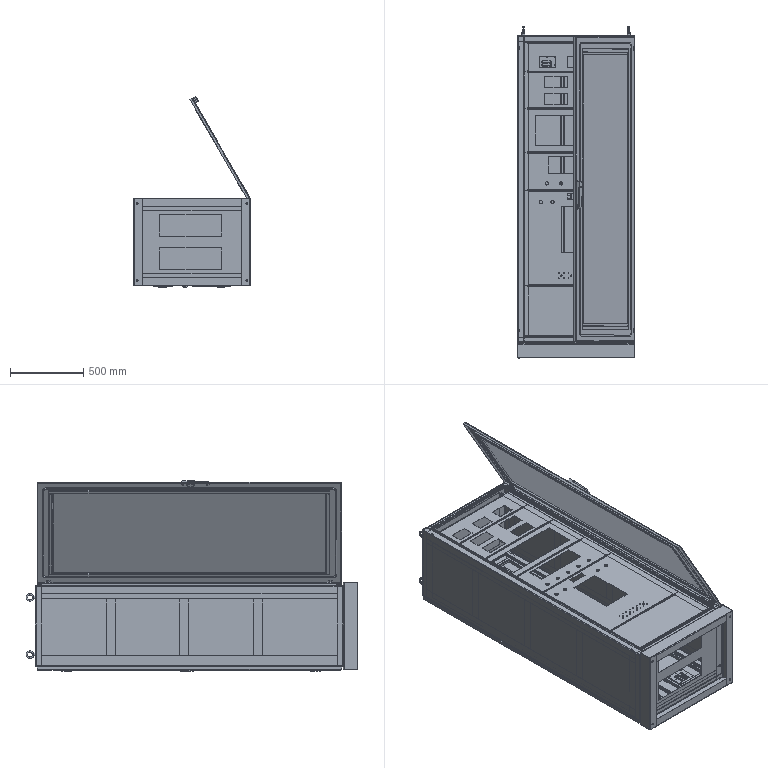Assembly | SolidWorks | mm | 69 component files | 69 solids | 2318 faces | box 801.74 x 2268 x 1304.71 mm | volume 31385291 mm3 | plane 1327 | cylinder 748 | torus 97 | sphere 64 | spline 46 | cone 36 | commonest cylinder face diameters 5 x100 7 x99 11 x91 4.5 x88 12.5 x48 3.2 x48 10 x48 2 x36
Bill of materials:
BaseFront-Rear | 2 |  | Long, thin-walled U-shaped channel with rounded inside bends. The base web runs past the ends of the two side walls at both ends.
BaseLeft-Right | 2 |  | Tall, thin-walled U or C channel with rounded bend corners. One side flange has two small round holes, one near each end.
Box | 2 | Plain Carbon Steel | Long, thin sheet panel with a C-shaped profile. A flat web has short flanges along both long edges, and each flange ends in a small hooked return lip.
CL201-M6-1 | 6 |  | Solid hinge-like block. An L-shaped body has two cylindrical knuckles with a shared pin bore at the two ends of one edge, a recessed gap between the knuckles, and a base leaf with two countersunk through holes and a chamfered edge.
CL201-M6-2 | 6 |  | Flat rectangular leaf plate with two round through holes. One edge thickens into a rounded knuckle lobe with a pin bore, as in a hinge leaf.
DoorLeftAndRightReinforcementBar | 6 | Malleable Cast Iron | Very long, slender, thin-walled channel. The end profile is a U shape with rounded bends and splayed straight legs.
DoorUpperAndLowerReinforcementBar | 2 | Malleable Cast Iron | Long, slender bar or channel. One end is rounded and the other end has a notched, C-like open profile. A recess or groove runs along its length.
FrontDoor | 1 | Malleable Cast Iron | Thin, flat rectangular frame plate with a large central rectangular cutout with small corner radii. A small rectangular slot and tiny holes sit near one long edge, and tiny holes are visible near the outer corners.
Glass | 1 | Plexiglas (TM) GS Acrylic Cast Sheet | Thin, plain, flat rectangular plate with no visible holes or cutouts.
MS829 | 1 | Cast Alloy Steel | Compact solid body with a stepped rectangular base. On one face is an elongated, tapered, raised paddle with a rounded end. On the opposite side is a protruding block with a cylindrical boss or pin. It looks like a lever or handle.
RubberPad | 1 | Silicone Rubber | Closed rectangular loop with rounded corners and a slender, thin cross-section, like a narrow rim or seal-shaped frame.
RearDoor1 | 1 | Malleable Cast Iron | Long, flat, thin rectangular sheet panel with shallow turned edges. One long edge has a small hooked return lip. Near each end is a small grid of perforation holes.
RearDoorUpperAndLowerReinforcementBar | 6 | Malleable Cast Iron | Long straight channel of uniform cross-section with an inverted-U profile (flat top, two parallel side legs, rounded outer corners), open along the bottom.
Vent | 4 | AISI 304 | Flat square plate with four parallel elongated louver-style formed openings in the middle and eight small round through-holes around the edge (corners and edge midpoints).
LiftingRingM12 | 4 |  | Ring-shaped eye with a round cross-section, joined to a cylindrical collar, with a smaller-diameter straight cylindrical shank coming out of the collar along the ring's radius.
LowerBaffle | 1 |  | Flat rectangular panel with two large rectangular cutouts stacked one above the other, four small holes near the side edges, and long formed flanges with short return lips along the top and bottom edges.
Panel1 | 1 | Malleable Cast Iron | Thin rectangular cover plate with three equal rectangular cutouts in a row, short downturned flanges along the two long edges, and small notches at the ends of the flanges.
Panel2 | 1 | Plain Carbon Steel | Thin rectangular cover plate with four rectangular cutouts in a 2x2 grid, short downturned flanges along the two long edges, and small notches where the flanges end.
Panel3 | 1 | Malleable Cast Iron | Thin rectangular frame-like plate with one large rectangular cutout in the middle, short downturned flanges along the two long edges, and notches where the flanges end.
Panel4 | 1 | Malleable Cast Iron | Thin rectangular cover plate with one rectangular cutout offset toward one long edge, a row of five equal round holes along the other long edge, and short downturned flanges along both long edges.
Panel5 | 1 | Malleable Cast Iron | Large thin rectangular plate with a tall rectangular cutout in the middle, a small rectangular slot above it, four round holes in a row near one edge, a pattern of small holes near the opposite edge, and very shallow downturned flanges along two edges.
Panel6 | 1 | Malleable Cast Iron | Plain thin rectangular plate with no openings, with short downturned flanges along the two long edges and notches where the flanges end.
PanelMountingBracket | 4 | Malleable Cast Iron | Long slender strip with an L-shaped (angle) cross-section, with a rounded inside bend between a wider leg and a narrower leg.
Lock818 | 1 |  | Small elongated part on a thin rectangular base plate. A raised block with rounded corners at one end slopes down to a long lower bar. A cylindrical post at the other end holds up a thin flat arm that runs back over the bar, parallel to it and spaced above it. A rounded protrusion sits on the underside.
RearDoor | 1 | Malleable Cast Iron | Long, narrow, thin rectangular plate or shallow tray with short edge returns along the perimeter, a rectangular slot near the middle of one long edge, and small groups of holes near each end.
SideBottomPlate | 2 | Plain Carbon Steel | Plain thin flat rectangular plate with no visible holes, cutouts or bends.
SideBottomPlateBracket | 6 | Malleable Cast Iron | Plain elongated flat rectangular strip or panel with no visible holes, cutouts or bends.
StiffenerPlate | 2 |  | Rectangular frame with a large central rectangular opening, narrow side bands each with two small round holes, and shallow return edges around the outer perimeter.
UpperBaffle | 1 |  | Flat rectangular panel with four small round corner holes. Top and bottom edges are formed into offset flanges with small lips, giving a C-like profile with hooked ends.
Mates:
1. coincident | StiffenerPlate-1 face at (-481.059, -83.54, -4140.526) dir (-1, 0, 0) | Box-1 face at (-481.059, 1976.46, -160.526) dir (1, 0, 0)
2. parallel | StiffenerPlate-1 face at (-4461.059, -83.54, 385.474) dir (0, 0, 1) | Box-1 face at (-433.059, 1976.46, -162.526) dir (0, 0, -1)
3. coincident | StiffenerPlate-1 face at (4294.941, -83.54, -160.526) dir (0, 0, -1) | Box-1 face at (-433.059, 1976.46, -160.526) dir (0, 0, 1)
4. coincident | StiffenerPlate-1 face at (214.919, -123.54, -84.019) dir (0, -1, 0) | Box-1 face at (-483.059, -123.54, -157.026) dir (0, -1, 0)
5. coincident | StiffenerPlate-1 face at (314.941, -83.54, 4365.474) dir (1, 0, 0) | Box-2 face at (314.941, -123.54, -160.526) dir (-1, 0, 0)
6. coincident | Box-1 face at (-433.059, 1976.46, -162.526) dir (0, 0, -1) | Box-2 face at (266.941, -123.54, -162.526) dir (0, 0, -1)
7. coincident | StiffenerPlate-1 face at (214.919, -123.54, -84.019) dir (0, -1, 0) | Box-2 face at (268.941, -123.54, -166.026) dir (0, -1, 0)
8. coincident | Box-1 face at (-481.059, 1976.46, -160.526) dir (1, 0, 0) | StiffenerPlate-2 face at (-481.059, 1936.46, 4365.474) dir (-1, 0, 0)
9. coincident | Box-2 face at (316.941, 1976.46, -157.026) dir (0, 1, 0) | StiffenerPlate-2 face at (214.919, 1976.46, 308.967) dir (0, 1, 0)
10. coincident | Box-2 face at (314.941, -123.54, 385.474) dir (0, 0, -1) | StiffenerPlate-2 face at (4294.941, 1936.46, 385.474) dir (0, 0, 1)
11. coincident | Box-1 face at (-481.059, 1976.46, 387.474) dir (0, 0, 1) | UpperBaffle-1 face at (316.941, 1930.46, 387.474) dir (0, 0, 1)
12. coincident | Box-1 face at (-483.059, 1976.46, -160.526) dir (-1, 0, 0) | UpperBaffle-1 face at (-483.059, 1972.96, -160.526) dir (-1, 0, 0)
13. coincident | Box-1 face at (-477.559, 1976.46, -162.526) dir (0, 1, 0) | UpperBaffle-1 face at (316.941, 1976.46, 387.474) dir (0, -1, 0)
14. concentric | UpperBaffle-1 face at (276.941, 1928.459, -82.526) dir (0, 1, 0) r 6.25 | LiftingRingM12-2 face at (276.941, 1953.46, -82.526) dir (0, 1, 0) r 6
15. coincident | UpperBaffle-1 face at (316.941, 1978.46, 387.474) dir (0, 1, 0) | LiftingRingM12-2 face at (276.941, 1978.46, -82.526) dir (0, -1, 0)
16. concentric | UpperBaffle-1 face at (276.941, 1928.459, 307.474) dir (0, 1, 0) r 6.25 | LiftingRingM12-1 face at (276.941, 1953.46, 307.474) dir (0, 1, 0) r 6
17. coincident | UpperBaffle-1 face at (316.941, 1978.46, 387.474) dir (0, 1, 0) | LiftingRingM12-1 face at (276.941, 1978.46, 307.474) dir (0, -1, 0)
18. concentric | UpperBaffle-1 face at (-443.059, 1928.459, 307.474) dir (0, 1, 0) r 6.25 | LiftingRingM12-4 face at (-443.059, 1953.46, 307.474) dir (0, 1, 0) r 6
19. coincident | UpperBaffle-1 face at (316.941, 1978.46, 387.474) dir (0, 1, 0) | LiftingRingM12-4 face at (-443.059, 1978.46, 307.474) dir (0, -1, 0)
20. concentric | UpperBaffle-1 face at (-443.059, 1928.459, -82.526) dir (0, 1, 0) r 6.25 | LiftingRingM12-3 face at (-443.059, 1953.46, -82.526) dir (0, 1, 0) r 6
21. coincident | UpperBaffle-1 face at (316.941, 1978.46, 387.474) dir (0, 1, 0) | LiftingRingM12-3 face at (-443.059, 1978.46, -82.526) dir (0, -1, 0)
22. coincident | Box-1 face at (-481.059, 1976.46, -160.526) dir (1, 0, 0) | PanelMountingBracket-1 face at (-481.059, 1936.46, 297.474) dir (-1, 0, 0)
23. coincident | Box-2 face at (314.941, -123.54, -160.526) dir (-1, 0, 0) | PanelMountingBracket-2 face at (314.941, -83.54, 297.474) dir (1, 0, 0)
24. parallel | Box-2 face at (266.941, -123.54, -162.526) dir (0, 0, -1) | PanelMountingBracket-2 face at (314.941, -83.54, 297.474) dir (0, 0, -1)
25. distance | PanelMountingBracket-2 face at (314.941, -83.54, 337.474) dir (0, 0, 1) | Box-2 face at (314.941, -123.54, 387.474) dir (0, 0, 1)
26. distance | Box-1 face at (-481.059, 1976.46, 387.474) dir (0, 0, 1) | PanelMountingBracket-1 face at (-481.059, 1936.46, 337.474) dir (0, 0, 1)
27. concentric | Box-2 face at (304.941, 1884.46, -168.89) dir (0, 0, 1) r 2.25 | CL201-M6-1-3 face at (304.941, 1884.46, 387.473) dir (0, 0, 1) r 2.25
28. coincident | Box-2 face at (314.941, -123.54, 387.474) dir (0, 0, 1) | CL201-M6-1-3 face at (314.728, 1914.46, 387.474) dir (0, 0, -1)
29. concentric | Box-2 face at (304.941, 1896.46, -168.89) dir (0, 0, 1) r 2.25 | CL201-M6-1-3 face at (304.941, 1896.46, 387.473) dir (0, 0, 1) r 2.25
30. coincident | Box-2 face at (314.941, -123.54, 387.474) dir (0, 0, 1) | CL201-M6-1-4 face at (314.728, -13.54, 387.474) dir (0, 0, -1)
31. concentric | Box-2 face at (304.941, -31.54, -168.89) dir (0, 0, 1) r 2.25 | CL201-M6-1-4 face at (304.941, -31.54, 387.473) dir (0, 0, 1) r 2.25
32. concentric | Box-2 face at (304.941, -43.54, -168.89) dir (0, 0, 1) r 2.25 | CL201-M6-1-4 face at (304.941, -43.54, 387.473) dir (0, 0, 1) r 2.25
33. coincident | FrontDoorAssembly-1/FrontDoor-1 face at (251.409, 1906.401, 517.975) dir (-0.866, 0, -0.5) | CL201-M6-2-4 face at (314.34, -25.04, 408.976) dir (0.866, 0, 0.5)
34. coincident | FrontDoorAssembly-1/FrontDoor-1 face at (251.409, 1906.401, 517.975) dir (-0.866, 0, -0.5) | CL201-M6-2-3 face at (314.34, 1902.96, 408.976) dir (0.866, 0, 0.5)
35. concentric | FrontDoorAssembly-1/FrontDoor-1 face at (310.858, -30.04, 419.009) dir (-0.866, 0, -0.5) r 1.6 | CL201-M6-2-4 face at (348.962, -30.04, 441.008) dir (-0.866, 0, -0.5) r 1.6
36. concentric | FrontDoorAssembly-1/FrontDoor-1 face at (310.858, -45.04, 419.009) dir (-0.866, 0, -0.5) r 1.6 | CL201-M6-2-4 face at (348.962, -45.04, 441.008) dir (-0.866, 0, -0.5) r 1.6
37. concentric | FrontDoorAssembly-1/FrontDoor-1 face at (310.858, 1897.96, 419.009) dir (-0.866, 0, -0.5) r 1.6 | CL201-M6-2-3 face at (348.962, 1897.96, 441.008) dir (-0.866, 0, -0.5) r 1.6
38. coincident | FrontDoorAssembly-1/FrontDoor-1 face at (310.858, 1882.96, 419.009) dir (-0.866, 0, -0.5) r 1.6 | CL201-M6-2-3 edge at (307.393, 1882.96, 417.008) dir (-0.866, 0, -0.5) r 1.6
39. concentric | CL201-M6-2-3 face at (311.742, 1902.96, 407.476) dir (0, -1, 0) r 1 | CL201-M6-1-3 face at (311.742, 1914.46, 407.476) dir (0, -1, 0) r 1
40. coincident | CL201-M6-2-3 face at (309.224, 1877.96, 409.744) dir (0, -1, 0) | CL201-M6-1-3 face at (301.242, 1877.96, 361.853) dir (0, 1, 0)
41. coincident | Box-2 face at (316.941, -123.54, -160.526) dir (1, 0, 0) | Base-1/BaseLeft-Right-1 face at (316.941, -225.54, 412.474) dir (1, 0, 0)
42. coincident | Base-1/BaseFront-Rear-1 face at (316.941, -125.54, -187.526) dir (0, 1, 0) | LowerBaffle-2 face at (316.941, -125.54, -162.526) dir (0, -1, 0)
43. coincident | StiffenerPlate-1 face at (4294.941, -83.54, -160.526) dir (0, 0, -1) | LowerBaffle-2 face at (316.941, -77.54, -160.526) dir (0, 0, 1)
44. coincident | Box-2 face at (316.941, -123.54, -160.526) dir (1, 0, 0) | LowerBaffle-2 face at (316.941, -120.04, -160.526) dir (1, 0, 0)
45. coincident | Box-2 face at (266.941, -123.54, -162.526) dir (0, 0, -1) | CL201-M6-1-8 face at (314.728, -61.54, -162.526) dir (0, 0, 1)
46. coincident | Box-2 face at (266.941, -123.54, -162.526) dir (0, 0, -1) | CL201-M6-1-6 face at (314.728, 1866.46, -162.526) dir (0, 0, 1)
47. coincident | Box-1 face at (-433.059, 1976.46, -162.526) dir (0, 0, -1) | CL201-M6-1-5 face at (-480.845, -13.54, -162.526) dir (0, 0, 1)
48. coincident | Box-1 face at (-433.059, 1976.46, -162.526) dir (0, 0, -1) | CL201-M6-1-7 face at (-480.845, 1914.46, -162.526) dir (0, 0, 1)
49. concentric | Box-2 face at (304.941, 1884.46, -168.89) dir (0, 0, 1) r 2.25 | CL201-M6-1-6 face at (304.941, 1884.46, -162.525) dir (0, 0, -1) r 2.25
50. concentric | Box-2 face at (304.941, 1896.46, -168.89) dir (0, 0, 1) r 2.25 | CL201-M6-1-6 face at (304.941, 1896.46, -162.525) dir (0, 0, -1) r 2.25
51. concentric | Box-2 face at (304.941, -43.54, -168.89) dir (0, 0, 1) r 2.25 | CL201-M6-1-8 face at (304.941, -43.54, -162.525) dir (0, 0, -1) r 2.25
52. concentric | Box-2 face at (304.941, -31.54, -168.89) dir (0, 0, 1) r 2.25 | CL201-M6-1-8 face at (304.941, -31.54, -162.525) dir (0, 0, -1) r 2.25
53. concentric | Box-1 face at (-471.059, 1896.46, -168.89) dir (0, 0, 1) r 2.25 | CL201-M6-1-7 face at (-471.059, 1896.46, -162.525) dir (0, 0, -1) r 2.25
54. concentric | Box-1 face at (-471.059, 1884.46, -168.89) dir (0, 0, 1) r 2.25 | CL201-M6-1-7 face at (-471.059, 1884.46, -162.525) dir (0, 0, -1) r 2.25
55. concentric | Box-1 face at (-471.059, -43.54, -168.89) dir (0, 0, 1) r 2.25 | CL201-M6-1-5 face at (-471.059, -43.54, -162.525) dir (0, 0, -1) r 2.25
56. concentric | Box-1 face at (-471.059, -31.54, -168.89) dir (0, 0, 1) r 2.25 | CL201-M6-1-5 face at (-471.059, -31.54, -162.525) dir (0, 0, -1) r 2.25
57. concentric | CL201-M6-1-5 face at (-477.86, -13.54, -182.528) dir (0, -1, 0) r 1 | CL201-M6-2-8 face at (-477.86, 1902.96, -182.528) dir (0, -1, 0) r 1
58. coincident | CL201-M6-2-8 face at (-474.637, 1902.96, -181.482) dir (0, 1, 0) | CL201-M6-1-7 face at (-467.36, 1902.96, -136.906) dir (0, -1, 0)
59. concentric | CL201-M6-2-6 face at (311.742, -50.04, -182.528) dir (0, 1, 0) r 1 | CL201-M6-1-8 face at (311.742, -61.54, -182.528) dir (0, 1, 0) r 1
60. coincident | CL201-M6-2-6 face at (308.516, -50.04, -181.49) dir (0, -1, 0) | CL201-M6-1-8 face at (301.242, -50.04, -136.906) dir (0, 1, 0)
61. coincident | CL201-M6-2-6 face at (311.749, -50.04, -185.528) dir (0.002502, 0, -1) | LeftRearDoor-1/RearDoor1-1 face at (185.888, -53.48, -185.843) dir (-0.002502, 0, 1)
62. concentric | CL201-M6-2-6 face at (301.434, -30.04, -231.554) dir (-0.002502, 0, 1) r 1.6 | LeftRearDoor-1/RearDoor1-1 face at (301.319, -30.04, -185.554) dir (0.002502, 0, -1) r 1.6
63. concentric | CL201-M6-2-6 face at (301.434, -30.04, -231.554) dir (-0.002502, 0, 1) r 1.6 | LeftRearDoor-1/RearDoor1-1 face at (301.319, -30.04, -185.554) dir (0.002502, 0, -1) r 1.6
64. concentric | CL201-M6-2-6 face at (301.434, -45.04, -231.554) dir (-0.002502, 0, 1) r 1.6 | LeftRearDoor-1/RearDoor1-1 face at (301.319, -45.04, -185.554) dir (0.002502, 0, -1) r 1.6
65. concentric | CL201-M6-1-5 face at (-477.86, -13.54, -182.528) dir (0, -1, 0) r 1 | CL201-M6-2-7 face at (-477.86, -25.04, -182.528) dir (0, -1, 0) r 1
66. coincident | CL201-M6-1-5 face at (-467.36, -25.04, -136.906) dir (0, -1, 0) | CL201-M6-2-7 face at (-474.637, -25.04, -181.482) dir (0, 1, 0)
67. coincident | CL201-M6-2-8 face at (-477.86, 1902.96, -185.528) dir (0, 0, -1) | RightRearDoor-1/RearDoor-1 face at (-351.997, 1906.401, -185.528) dir (0, 0, 1)
68. concentric | CL201-M6-2-8 face at (-467.43, 1897.96, -231.528) dir (0, 0, 1) r 1.6 | RightRearDoor-1/RearDoor-1 face at (-467.43, 1897.96, -167.527) dir (0, 0, -1) r 1.6
69. concentric | CL201-M6-2-8 face at (-467.43, 1882.96, -231.528) dir (0, 0, 1) r 1.6 | RightRearDoor-1/RearDoor-1 face at (-467.43, 1882.96, -167.527) dir (0, 0, -1) r 1.6
70. coincident | Panel6-1 face at (-384.146, 150.197, 339.474) dir (0, 0, 1) | Panel5-2 face at (-364.146, 800.197, 339.474) dir (0, 0, 1)
71. coincident | Panel6-1 face at (-384.146, 268.46, 339.474) dir (0, 1, 0) | Panel5-2 face at (-364.146, 268.46, 339.474) dir (0, -1, 0)
72. coincident | Panel5-2 face at (-364.146, 918.46, 339.474) dir (0, 1, 0) | Panel4-2 face at (-344.146, 918.46, 339.474) dir (0, -1, 0)
73. coincident | Panel5-2 face at (-364.146, 800.197, 339.474) dir (0, 0, 1) | Panel4-2 face at (-344.146, 1060.197, 339.474) dir (0, 0, 1)
74. coincident | Panel4-2 face at (-344.146, 1178.46, 339.474) dir (0, 1, 0) | Panel3-2 face at (-384.146, 1178.46, 339.474) dir (0, -1, 0)
75. coincident | Panel4-2 face at (-344.146, 1060.197, 339.474) dir (0, 0, 1) | Panel3-2 face at (-384.146, 1360.197, 339.474) dir (0, 0, 1)
76. coincident | Panel4-2 face at (288.941, 1178.46, 337.474) dir (1, 0, 0) | Panel3-2 face at (288.941, 1478.46, 337.474) dir (1, 0, 0)
77. coincident | Panel3-2 face at (-384.146, 1360.197, 339.474) dir (0, 0, 1) | Panel2-2 face at (-344.146, 1650.197, 339.474) dir (0, 0, 1)
78. coincident | Panel3-2 face at (288.941, 1478.46, 337.474) dir (1, 0, 0) | Panel2-2 face at (288.941, 1728.46, 337.474) dir (1, 0, 0)
79. coincident | Panel3-2 face at (-384.146, 1478.46, 339.474) dir (0, 1, 0) | Panel2-2 face at (-344.146, 1478.46, 339.474) dir (0, -1, 0)
80. coincident | Panel2-2 face at (-344.146, 1650.197, 339.474) dir (0, 0, 1) | Panel1-2 face at (-344.146, 1940.197, 339.474) dir (0, 0, 1)
81. coincident | Panel2-2 face at (-344.146, 1728.46, 339.474) dir (0, 1, 0) | Panel1-2 face at (-344.146, 1728.46, 339.474) dir (0, -1, 0)
82. coincident | Panel2-2 face at (288.941, 1728.46, 337.474) dir (1, 0, 0) | Panel1-2 face at (288.941, 1928.46, 337.474) dir (1, 0, 0)
83. coincident | Box-2 face at (314.941, -123.54, -160.526) dir (-1, 0, 0) | PanelMountingBracket-3 face at (314.941, -83.54, -160.526) dir (1, 0, 0)
84. coincident | Box-2 face at (266.941, -123.54, -160.526) dir (0, 0, 1) | PanelMountingBracket-3 face at (274.941, -83.54, -160.526) dir (0, 0, -1)
85. coincident | Box-1 face at (-481.059, 1976.46, -160.526) dir (1, 0, 0) | PanelMountingBracket-4 face at (-481.059, 1936.46, -160.526) dir (-1, 0, 0)
86. coincident | Box-1 face at (-433.059, 1976.46, -160.526) dir (0, 0, 1) | PanelMountingBracket-4 face at (-441.059, 1936.46, -160.526) dir (0, 0, -1)
87. coincident | Box-1 face at (-481.059, 1976.46, -160.526) dir (1, 0, 0) | SideBottomPlateBracket-5 face at (-481.059, 488.96, -90.526) dir (-1, 0, 0)
88. coincident | SideBottomPlateBracket-5 face at (-563.101, 452.513, -90.526) dir (0, 0, -1) | PanelMountingBracket-4 face at (-479.059, 1936.46, -90.526) dir (0, 0, 1)
89. coincident | SideBottomPlateBracket-4 face at (-563.101, 955.013, -90.526) dir (0, 0, -1) | PanelMountingBracket-4 face at (-479.059, 1936.46, -90.526) dir (0, 0, 1)
90. coincident | SideBottomPlateBracket-6 face at (-563.101, 1457.513, -90.526) dir (0, 0, -1) | PanelMountingBracket-4 face at (-479.059, 1936.46, -90.526) dir (0, 0, 1)
91. coincident | SideBottomPlateBracket-3 face at (396.983, 452.513, -90.526) dir (0, 0, -1) | PanelMountingBracket-3 face at (312.941, -83.54, -90.526) dir (0, 0, 1)
92. coincident | SideBottomPlateBracket-1 face at (396.983, 955.013, -90.526) dir (0, 0, -1) | PanelMountingBracket-3 face at (312.941, -83.54, -90.526) dir (0, 0, 1)
93. coincident | SideBottomPlateBracket-2 face at (396.983, 1457.513, -90.526) dir (0, 0, -1) | PanelMountingBracket-3 face at (312.941, -83.54, -90.526) dir (0, 0, 1)
94. coincident | Box-1 face at (-481.059, 1976.46, -160.526) dir (1, 0, 0) | SideBottomPlateBracket-4 face at (-481.059, 991.46, -90.526) dir (-1, 0, 0)
95. coincident | Box-1 face at (-481.059, 1976.46, -160.526) dir (1, 0, 0) | SideBottomPlateBracket-6 face at (-481.059, 1493.96, -90.526) dir (-1, 0, 0)
96. coincident | Box-2 face at (314.941, -123.54, -160.526) dir (-1, 0, 0) | SideBottomPlateBracket-2 face at (314.941, 1493.96, 297.474) dir (1, 0, 0)
97. coincident | Box-2 face at (314.941, -123.54, -160.526) dir (-1, 0, 0) | SideBottomPlateBracket-1 face at (314.941, 991.46, 297.474) dir (1, 0, 0)
98. coincident | Box-2 face at (314.941, -123.54, -160.526) dir (-1, 0, 0) | SideBottomPlateBracket-3 face at (314.941, 488.96, 297.474) dir (1, 0, 0)
99. distance | StiffenerPlate-2 face at (-481.059, 1936.46, 4365.474) dir (0, -1, 0) | SideBottomPlateBracket-6 face at (-481.059, 1433.96, -90.526) dir (0, -1, 0)
100. distance | SideBottomPlateBracket-4 face at (-481.059, 931.46, -90.526) dir (0, -1, 0) | StiffenerPlate-2 face at (-481.059, 1936.46, 4365.474) dir (0, -1, 0)
101. distance | StiffenerPlate-2 face at (-481.059, 1936.46, 4365.474) dir (0, -1, 0) | SideBottomPlateBracket-5 face at (-481.059, 428.96, -90.526) dir (0, -1, 0)
102. distance | StiffenerPlate-2 face at (314.941, 1936.46, -4140.526) dir (0, -1, 0) | SideBottomPlateBracket-2 face at (314.941, 1433.96, 297.474) dir (0, -1, 0)
103. distance | StiffenerPlate-2 face at (314.941, 1936.46, -4140.526) dir (0, -1, 0) | SideBottomPlateBracket-1 face at (314.941, 931.46, 297.474) dir (0, -1, 0)
104. distance | StiffenerPlate-2 face at (314.941, 1936.46, -4140.526) dir (0, -1, 0) | SideBottomPlateBracket-3 face at (314.941, 428.96, 297.474) dir (0, -1, 0)
105. distance | UpperBaffle-1 face at (316.941, 1976.46, 387.474) dir (0, -1, 0) | Panel1-2 edge at (-403.559, 1926.46, 319.474) dir (1, 0, 0)
106. coincident | CL201-M6-2-5 face at (311.742, 1877.96, -182.528) dir (0, 1, 0) r 1 | CL201-M6-1-6 edge at (311.742, 1914.46, -182.528) dir (0, -1, 0) r 1
107. coincident | CL201-M6-2-5 face at (308.516, 1902.96, -181.49) dir (0, 1, 0) | CL201-M6-1-6 face at (301.242, 1902.96, -136.906) dir (0, -1, 0)
108. coincident | CL201-M6-2-5 face at (311.749, 1877.96, -185.528) dir (0.002502, 0, -1) | LeftRearDoor-1/RearDoor1-1 face at (185.888, -53.48, -185.843) dir (-0.002502, 0, 1)
109. coincident | CL201-M6-2-7 face at (-477.86, -25.04, -185.528) dir (0, 0, -1) | RightRearDoor-1/RearDoor-1 face at (-351.997, 1906.401, -185.528) dir (0, 0, 1)
110. coincident | SideBottomPlateBracket-6 face at (-479.059, 1493.96, -90.526) dir (1, 0, 0) | SideBottomPlate-1 face at (-479.059, 1823.112, -40.634) dir (-1, 0, 0)
111. distance | SideBottomPlate-1 face at (-477.059, 1878.46, -132.526) dir (0, 0, -1) | Box-1 face at (-433.059, 1976.46, -162.526) dir (0, 0, -1)
112. distance | SideBottomPlate-1 face at (-477.059, 1878.46, -132.526) dir (0, 1, 0) | UpperBaffle-1 face at (316.941, 1978.46, 387.474) dir (0, 1, 0)
113. coincident | SideBottomPlateBracket-3 face at (312.941, 488.96, 297.474) dir (-1, 0, 0) | SideBottomPlate-2 face at (312.941, 1823.112, 235.581) dir (1, 0, 0)
114. distance | SideBottomPlate-2 face at (310.941, 1878.46, -132.526) dir (0, 0, -1) | Box-2 face at (266.941, -123.54, -162.526) dir (0, 0, -1)
115. distance | SideBottomPlate-2 face at (310.941, 1878.46, 327.474) dir (0, 1, 0) | UpperBaffle-1 face at (316.941, 1978.46, 387.474) dir (0, 1, 0)
116. distance | Base-1/BaseFront-Rear-2 face at (-483.059, -225.54, 412.474) dir (0, 0, 1) | Box-1 face at (-481.059, 1976.46, 387.474) dir (0, 0, 1)
117. coincident | PanelMountingBracket-1 face at (-481.059, 1936.46, 337.474) dir (0, 0, 1) | Panel6-1 face at (-384.146, 150.197, 337.474) dir (0, 0, -1)
118. parallel | Box-1 face at (-483.059, 1976.46, -160.526) dir (-1, 0, 0) | Panel2-2 face at (-456.059, 1728.46, 337.474) dir (-1, 0, 0)
119. distance | Box-1 face at (-481.059, 1976.46, -160.526) dir (1, 0, 0) | Panel2-2 face at (-456.059, 1728.46, 337.474) dir (-1, 0, 0)
120. parallel | UpperBaffle-1 face at (316.941, 1978.46, -162.526) dir (0, 0, -1) | RightRearDoor-1/RearDoor-1 face at (-351.997, 1906.401, -187.528) dir (0, 0, -1)
121. coincident | Panel6-1 face at (288.941, 268.46, 337.474) dir (1, 0, 0) | Panel5-2 face at (288.941, 918.46, 329.474) dir (1, 0, 0)
122. coincident | Panel5-2 face at (288.941, 918.46, 329.474) dir (1, 0, 0) | Panel4-2 face at (288.941, 1178.46, 337.474) dir (1, 0, 0)
123. distance | UpperBaffle-1 face at (316.941, 1976.46, 387.474) dir (0, -1, 0) | PanelMountingBracket-1 face at (-475.559, 1936.46, 335.474) dir (0, 1, 0)
124. distance | UpperBaffle-1 face at (316.941, 1976.46, 387.474) dir (0, -1, 0) | PanelMountingBracket-2 face at (312.941, 1936.46, 331.974) dir (0, 1, 0)
125. distance | StiffenerPlate-1 face at (214.919, -123.54, -84.019) dir (0, -1, 0) | PanelMountingBracket-3 face at (309.441, -83.54, -155.026) dir (0, -1, 0)
126. distance | Box-1 face at (-477.559, -123.54, 387.474) dir (0, -1, 0) | PanelMountingBracket-4 face at (-475.559, -83.54, -158.526) dir (0, -1, 0)
127. distance | StiffenerPlate-1 edge at (259.941, -123.54, -105.526) dir (-1, 0, 0) | Base-1/BaseFront-Rear-2 face at (-483.059, -125.54, 412.474) dir (0, 1, 0)
128. coincident | BaseLeft-Right-1 face at (-198.927, 256.734, 189.72) dir (1, 0, 0) | BaseFront-Rear-2 face at (-198.927, 256.734, -610.28) dir (1, 0, 0)
129. coincident | BaseLeft-Right-1 face at (-198.927, 256.734, 189.72) dir (1, 0, 0) | BaseFront-Rear-1 face at (-198.927, -343.266, 189.72) dir (1, 0, 0)
130. coincident | BaseLeft-Right-2 face at (-198.927, -343.266, -610.28) dir (1, 0, 0) | BaseFront-Rear-1 face at (-198.927, -343.266, 189.72) dir (1, 0, 0)
131. coincident | BaseLeft-Right-2 face at (-198.927, -343.266, -610.28) dir (1, 0, 0) | BaseFront-Rear-2 face at (-198.927, 256.734, -610.28) dir (1, 0, 0)
132. coincident | BaseLeft-Right-2 face at (-200.927, -343.266, -550.28) dir (0, 0, 1) | BaseFront-Rear-2 face at (-200.927, 256.734, -550.28) dir (0, 0, -1)
133. coincident | BaseLeft-Right-1 face at (-298.927, 256.734, 129.72) dir (0, 0, -1) | BaseFront-Rear-2 face at (-296.927, 196.734, 129.72) dir (0, 0, 1)
134. coincident | BaseLeft-Right-1 face at (-293.427, 256.734, 187.72) dir (0, 1, 0) | BaseFront-Rear-2 face at (-298.927, 256.734, -610.28) dir (0, 1, 0)
135. coincident | BaseLeft-Right-2 face at (-298.927, -343.266, -550.28) dir (-1, 0, 0) | BaseFront-Rear-1 face at (-298.927, -283.266, 189.72) dir (-1, 0, 0)
136. coincident | BaseLeft-Right-2 face at (-298.927, -343.266, -610.28) dir (0, 0, -1) | BaseFront-Rear-1 face at (-296.927, -337.766, -610.28) dir (0, 0, -1)
137. coincident | BaseLeft-Right-1 face at (-204.427, -343.266, 184.22) dir (0, -1, 0) | BaseFront-Rear-1 face at (-298.927, -343.266, 189.72) dir (0, -1, 0)
138. coincident | BaseLeft-Right-2 face at (-204.427, 256.734, -608.28) dir (0, 1, 0) | BaseFront-Rear-2 face at (-298.927, 256.734, -610.28) dir (0, 1, 0)
139. coincident | FrontDoor-1 face at (-893.651, 893.809, -5.5) dir (0, 0, 1) | DoorLeftAndRightReinforcementBar-2 face at (-310.584, 873.869, -5.5) dir (0, 0, -1)
140. coincident | FrontDoor-1 face at (-893.651, 893.809, -5.5) dir (0, 0, 1) | DoorLeftAndRightReinforcementBar-1 face at (-965.584, 873.869, -5.5) dir (0, 0, -1)
141. distance | DoorLeftAndRightReinforcementBar-2 face at (-285.584, 873.869, -5.5) dir (1, 0, 0) | FrontDoor-1 face at (-225.584, 11353.869, 12.5) dir (1, 0, 0)
142. distance | DoorLeftAndRightReinforcementBar-1 face at (-965.584, 873.869, 14.5) dir (-1, 0, 0) | FrontDoor-1 face at (-1025.584, -11526.131, 12.5) dir (-1, 0, 0)
143. coincident | FrontDoor-1 face at (-893.651, 893.809, -5.5) dir (0, 0, 1) | DoorUpperAndLowerReinforcementBar-1 face at (-940.584, 848.869, -5.5) dir (0, 0, -1)
144. coincident | FrontDoor-1 face at (-893.651, 893.809, -5.5) dir (0, 0, 1) | DoorUpperAndLowerReinforcementBar-2 face at (-940.584, -1046.131, -5.5) dir (0, 0, -1)
145. distance | FrontDoor-1 face at (10174.416, -1126.131, 12.5) dir (0, -1, 0) | DoorUpperAndLowerReinforcementBar-2 face at (-940.584, -1046.131, 14.5) dir (0, -1, 0)
146. distance | DoorUpperAndLowerReinforcementBar-1 face at (-940.584, 873.869, -5.5) dir (0, 1, 0) | FrontDoor-1 face at (-11425.584, 953.869, 12.5) dir (0, 1, 0)
147. coincident | DoorUpperAndLowerReinforcementBar-1 face at (-940.584, 873.869, -5.5) dir (0, 1, 0) | DoorLeftAndRightReinforcementBar-2 face at (-305.084, 873.869, 12.5) dir (0, 1, 0)
148. coincident | DoorUpperAndLowerReinforcementBar-1 face at (-940.584, 873.869, -5.5) dir (0, 1, 0) | DoorLeftAndRightReinforcementBar-1 face at (-960.084, 873.869, 9) dir (0, 1, 0)
149. coincident | DoorUpperAndLowerReinforcementBar-1 face at (-310.584, 868.369, 12.5) dir (1, 0, 0) | DoorLeftAndRightReinforcementBar-2 face at (-310.584, 873.869, 14.5) dir (-1, 0, 0)
150. coincident | DoorUpperAndLowerReinforcementBar-2 face at (-940.584, -1040.631, 9) dir (-1, 0, 0) | DoorLeftAndRightReinforcementBar-1 face at (-940.584, 873.869, -5.5) dir (1, 0, 0)
151. coincident | FrontDoor-1 face at (-893.651, 893.809, -5.5) dir (0, 0, 1) | RubberPad-1 face at (-971.446, -1067.422, -5.5) dir (0, 0, -1)
152. parallel | FrontDoor-1 face at (-1025.584, -11526.131, 12.5) dir (-1, 0, 0) | RubberPad-1 edge at (-981.446, 892.578, -5.5) dir (0, -1, 0)
153. coincident | FrontDoor-1 face at (-893.651, 893.809, -7.5) dir (0, 0, -1) | MS829-1 face at (-230.084, -29.431, -7.5) dir (0, 0, 1)
154. concentric | FrontDoor-1 face at (-247.584, -41.131, 12.501) dir (0, 0, -1) r 2.75 | MS829-1 face at (-247.584, -41.131, 2.5) dir (0, 0, -1) r 2.75
155. coincident | FrontDoor-1 face at (-893.651, 893.809, -5.5) dir (0, 0, 1) | Glass-1 face at (-801.689, 795.978, -5.5) dir (0, 0, -1)
156. distance | DoorUpperAndLowerReinforcementBar-2 face at (-940.584, -1021.131, -5.5) dir (0, 1, 0) | Glass-1 face at (-935.584, -1016.131, -5.5) dir (0, -1, 0)
157. distance | DoorLeftAndRightReinforcementBar-1 face at (-940.584, 873.869, -5.5) dir (1, 0, 0) | Glass-1 face at (-935.584, 843.869, -5.5) dir (-1, 0, 0)
158. coincident | RearDoor1-1 face at (-676.222, 877.442, 378.385) dir (0, 0, 1) | DoorLeftAndRightReinforcementBar-2 face at (-513.155, 857.501, 378.385) dir (0, 0, -1)
159. coincident | RearDoor1-1 face at (-676.222, 877.442, 378.385) dir (0, 0, 1) | DoorLeftAndRightReinforcementBar-1 face at (-753.155, 857.501, 378.385) dir (0, 0, -1)
160. distance | DoorLeftAndRightReinforcementBar-2 face at (-488.155, 857.501, 378.385) dir (1, 0, 0) | RearDoor1-1 face at (-408.155, 11337.501, 396.385) dir (1, 0, 0)
161. distance | DoorLeftAndRightReinforcementBar-1 face at (-753.155, 857.501, 398.385) dir (-1, 0, 0) | RearDoor1-1 face at (-808.155, -11542.499, 396.385) dir (-1, 0, 0)
162. distance | DoorLeftAndRightReinforcementBar-1 face at (-733.655, -1062.499, 396.385) dir (0, -1, 0) | RearDoor1-1 face at (9991.845, -1142.499, 396.385) dir (0, -1, 0)
163. distance | DoorLeftAndRightReinforcementBar-2 face at (-493.655, -1062.499, 396.385) dir (0, -1, 0) | RearDoor1-1 edge at (-410.331, -1142.499, 381.885) dir (-1, 0, 0)
164. coincident | RearDoor1-1 face at (-676.222, 877.442, 378.385) dir (0, 0, 1) | RearDoorUpperAndLowerReinforcementBar-1 face at (-728.155, -1062.499, 378.385) dir (0, 0, -1)
165. coincident | RearDoor1-1 face at (-676.222, 877.442, 378.385) dir (0, 0, 1) | RearDoorUpperAndLowerReinforcementBar-3 face at (-728.155, -112.499, 378.385) dir (0, 0, -1)
166. coincident | RearDoor1-1 face at (-676.222, 877.442, 378.385) dir (0, 0, 1) | RearDoorUpperAndLowerReinforcementBar-2 face at (-728.155, 832.501, 378.385) dir (0, 0, -1)
167. coincident | RearDoorUpperAndLowerReinforcementBar-3 face at (-513.155, -92.999, 396.385) dir (1, 0, 0) | DoorLeftAndRightReinforcementBar-2 face at (-513.155, 857.501, 398.385) dir (-1, 0, 0)
168. coincident | RearDoorUpperAndLowerReinforcementBar-1 face at (-513.155, -1042.999, 396.385) dir (1, 0, 0) | DoorLeftAndRightReinforcementBar-2 face at (-513.155, 857.501, 398.385) dir (-1, 0, 0)
169. coincident | RearDoorUpperAndLowerReinforcementBar-2 face at (-513.155, 852.001, 396.385) dir (1, 0, 0) | DoorLeftAndRightReinforcementBar-2 face at (-513.155, 857.501, 398.385) dir (-1, 0, 0)
170. coincident | RearDoorUpperAndLowerReinforcementBar-1 face at (-728.155, -1062.499, 398.385) dir (0, -1, 0) | DoorLeftAndRightReinforcementBar-2 face at (-493.655, -1062.499, 396.385) dir (0, -1, 0)
171. coincident | RearDoorUpperAndLowerReinforcementBar-2 face at (-728.155, 857.501, 378.385) dir (0, 1, 0) | DoorLeftAndRightReinforcementBar-2 face at (-507.655, 857.501, 396.385) dir (0, 1, 0)
172. distance | RearDoorUpperAndLowerReinforcementBar-2 face at (-728.155, 857.501, 378.385) dir (0, 1, 0) | RearDoorUpperAndLowerReinforcementBar-3 face at (-728.155, -112.499, 398.385) dir (0, -1, 0)
173. coincident | RearDoor1-1 face at (-676.222, 877.442, 376.385) dir (0, 0, -1) | Vent-1 face at (-605.655, 750.001, 376.385) dir (0, 0, 1)
174. coincident | RearDoor1-1 face at (-676.222, 877.442, 376.385) dir (0, 0, -1) | Vent-2 face at (-606.007, -955.351, 376.385) dir (0, 0, 1)
175. concentric | RearDoor1-1 face at (-553.655, -1007.499, 398.386) dir (0, 0, -1) r 2.5 | Vent-2 face at (-553.655, -1007.499, 376.385) dir (0, 0, -1) r 2.5
176. concentric | RearDoor1-1 face at (-553.655, 697.501, 398.386) dir (0, 0, -1) r 2.5 | Vent-1 face at (-553.655, 697.501, 376.385) dir (0, 0, -1) r 2.5
177. parallel | RearDoor1-1 face at (-808.155, -11542.499, 396.385) dir (-1, 0, 0) | Vent-1 face at (-670.655, 685.001, 376.385) dir (-1, 0, 0)
178. coincident | RearDoor-1 face at (-952.894, 877.647, 528.407) dir (0, 0, 1) | DoorLeftAndRightReinforcementBar-2 face at (-789.827, 857.707, 528.407) dir (0, 0, -1)
179. coincident | RearDoor-1 face at (-952.894, 877.647, 528.407) dir (0, 0, 1) | DoorLeftAndRightReinforcementBar-1 face at (-1006.827, 857.707, 528.407) dir (0, 0, -1)
180. distance | DoorLeftAndRightReinforcementBar-2 face at (-764.827, 857.707, 528.407) dir (1, 0, 0) | RearDoor-1 face at (-684.827, 11337.707, 546.407) dir (1, 0, 0)
181. distance | DoorLeftAndRightReinforcementBar-1 face at (-1029.827, 857.707, 548.407) dir (-1, 0, 0) | RearDoor-1 face at (-1084.827, -11542.293, 546.407) dir (-1, 0, 0)
182. coincident | RearDoor-1 face at (-952.894, 877.647, 528.407) dir (0, 0, 1) | RearDoorUpperAndLowerReinforcementBar-2 face at (-1004.827, -1062.293, 528.407) dir (0, 0, -1)
183. coincident | RearDoor-1 face at (-952.894, 877.647, 528.407) dir (0, 0, 1) | RearDoorUpperAndLowerReinforcementBar-1 face at (-1004.827, 832.707, 528.407) dir (0, 0, -1)
184. coincident | DoorLeftAndRightReinforcementBar-1 face at (-1004.827, 857.707, 528.407) dir (1, 0, 0) | RearDoorUpperAndLowerReinforcementBar-1 face at (-1004.827, 838.207, 542.907) dir (-1, 0, 0)
185. coincident | DoorLeftAndRightReinforcementBar-1 face at (-1024.327, 857.707, 542.907) dir (0, 1, 0) | RearDoorUpperAndLowerReinforcementBar-1 face at (-1004.827, 857.707, 528.407) dir (0, 1, 0)
186. coincident | DoorLeftAndRightReinforcementBar-2 face at (-789.827, 857.707, 548.407) dir (-1, 0, 0) | RearDoorUpperAndLowerReinforcementBar-2 face at (-789.827, -1056.793, 542.907) dir (1, 0, 0)
187. coincident | DoorLeftAndRightReinforcementBar-2 face at (-784.327, -1062.293, 542.907) dir (0, -1, 0) | RearDoorUpperAndLowerReinforcementBar-2 face at (-1004.827, -1062.293, 548.407) dir (0, -1, 0)
188. distance | DoorLeftAndRightReinforcementBar-1 face at (-1010.327, -1062.293, 546.407) dir (0, -1, 0) | RearDoor-1 face at (9715.173, -1142.293, 546.407) dir (0, -1, 0)
189. distance | DoorLeftAndRightReinforcementBar-2 face at (-784.327, -1062.293, 542.907) dir (0, -1, 0) | RearDoor-1 face at (9715.173, -1142.293, 546.407) dir (0, -1, 0)
190. coincident | RearDoor-1 face at (-952.894, 877.647, 528.407) dir (0, 0, 1) | RearDoorUpperAndLowerReinforcementBar-3 face at (-1004.827, -112.293, 528.407) dir (0, 0, -1)
191. coincident | DoorLeftAndRightReinforcementBar-2 face at (-789.827, 857.707, 548.407) dir (-1, 0, 0) | RearDoorUpperAndLowerReinforcementBar-3 face at (-789.827, -92.793, 546.407) dir (1, 0, 0)
192. distance | RearDoorUpperAndLowerReinforcementBar-1 face at (-1004.827, 857.707, 528.407) dir (0, 1, 0) | RearDoorUpperAndLowerReinforcementBar-3 face at (-1004.827, -112.293, 548.407) dir (0, -1, 0)
193. coincident | RearDoor-1 face at (-952.894, 877.647, 526.407) dir (0, 0, -1) | Vent-1 face at (-883.327, 750.207, 526.407) dir (0, 0, 1)
194. concentric | RearDoor-1 face at (-935.327, 802.707, 536.407) dir (0, 0, -1) r 2.5 | Vent-1 face at (-935.327, 802.707, 526.407) dir (0, 0, -1) r 2.5
195. concentric | RearDoor-1 face at (-935.327, 697.707, 536.407) dir (0, 0, -1) r 2.5 | Vent-1 face at (-935.327, 697.707, 526.407) dir (0, 0, -1) r 2.5
196. coincident | RearDoor-1 face at (-952.894, 877.647, 526.407) dir (0, 0, -1) | Vent-2 face at (-882.327, -954.793, 526.407) dir (0, 0, 1)
197. concentric | RearDoor-1 face at (-830.327, -1007.293, 536.407) dir (0, 0, -1) r 2.5 | Vent-2 face at (-830.327, -1007.293, 526.407) dir (0, 0, -1) r 2.5
198. concentric | RearDoor-1 face at (-830.327, -902.293, 536.407) dir (0, 0, -1) r 2.5 | Vent-2 face at (-830.327, -902.293, 526.407) dir (0, 0, -1) r 2.5
199. coincident | RearDoor-1 face at (-952.894, 877.647, 526.407) dir (0, 0, -1) | Lock818-1 face at (-736.327, -69.427, 526.407) dir (0, 0, 1)
200. coincident | RearDoor-1 face at (-722.327, -34.793, 546.408) dir (0, -1, 0) | Lock818-1 face at (-722.327, -34.793, 556.407) dir (0, 1, 0)
201. coincident | RearDoor-1 face at (-722.327, -34.793, 546.408) dir (-1, 0, 0) | Lock818-1 face at (-722.327, -164.793, 556.407) dir (1, 0, 0)